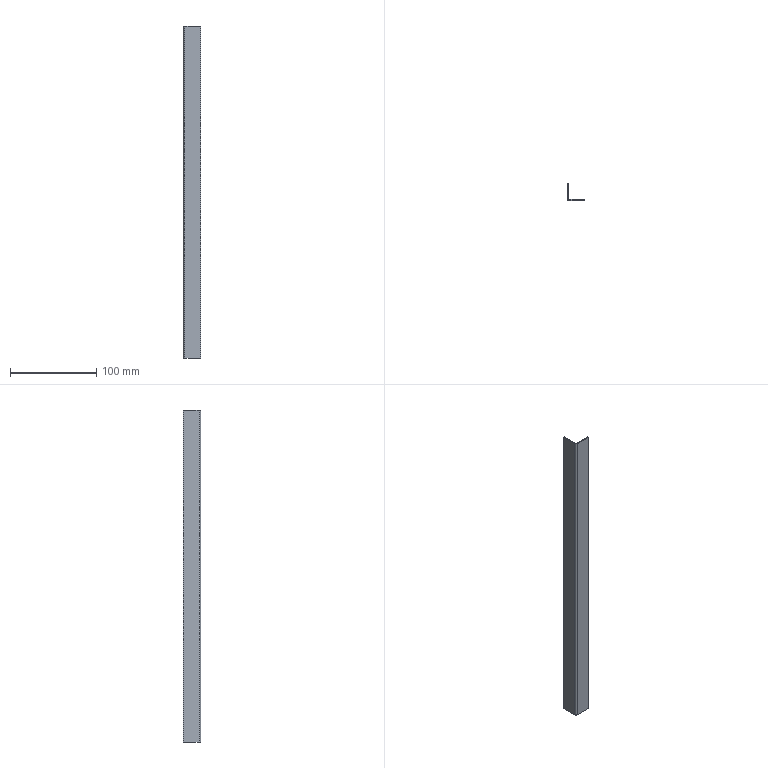Component | SolidWorks | CCQ-1.1-1AngleIron-2 | 1 solid | 14 faces | volume 14811 mm3 | plane 12 | cylinder 2 | commonest cylinder face diameters 1.473 x1 3.473 x1 | material 304